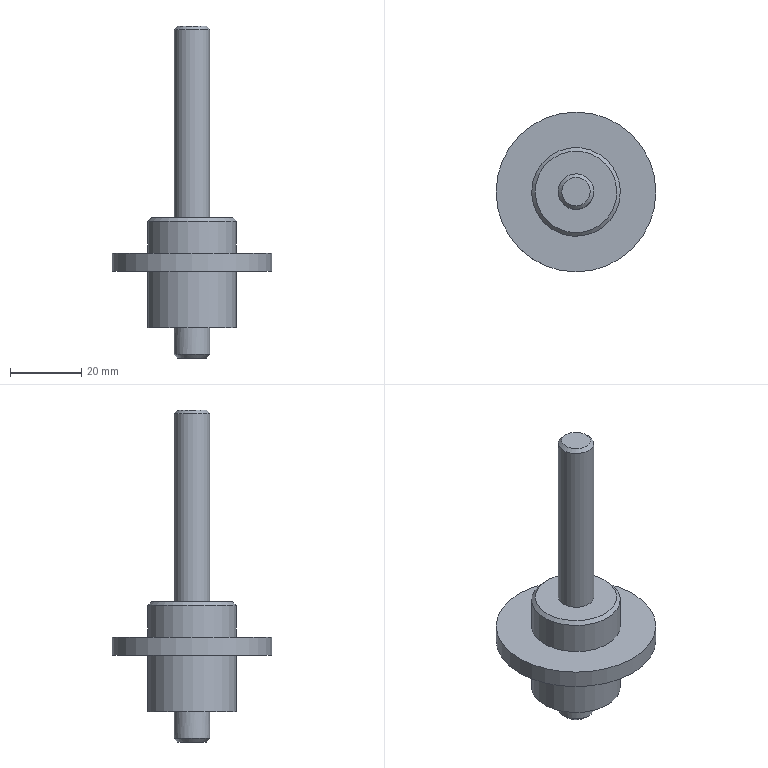Component | NX | MANDREL | 1 solid | 14 faces | box 45 x 45 x 93.5 mm | volume 25556 mm3 | plane 6 | cylinder 5 | cone 3 | commonest cylinder face diameters 25 x2 10 x2 45 x1
STEP:
#1=CARTESIAN_POINT('',(0.,0.,0.));
#2=DIRECTION('',(0.,0.,1.));
#3=DIRECTION('',(1.,0.,0.));
#4=AXIS2_PLACEMENT_3D('',#1,#2,#3);
#5=CARTESIAN_POINT('',(94.615,72.307,11.));
#6=VERTEX_POINT('',#5);
#7=CARTESIAN_POINT('',(89.996,70.391,11.));
#8=DIRECTION('',(0.,0.,-1.));
#9=DIRECTION('',(0.9237,0.383,0.));
#10=AXIS2_PLACEMENT_3D('',#7,#8,#9);
#11=CIRCLE('',#10,5.);
#12=CARTESIAN_POINT('',(89.996,70.391,11.));
#13=DIRECTION('',(0.,0.,1.));
#14=DIRECTION('',(0.383,-0.9237,0.));
#15=AXIS2_PLACEMENT_3D('',#12,#13,#14);
#16=PLANE('',#15);
#17=CARTESIAN_POINT('',(-0.,5.));
#18=CARTESIAN_POINT('',(8.66,5.));
#19=CARTESIAN_POINT('',(4.33,-2.5));
#20=CARTESIAN_POINT('',(0.,-10.));
#21=CARTESIAN_POINT('',(-4.33,-2.5));
#22=CARTESIAN_POINT('',(-8.66,5.));
#23=CARTESIAN_POINT('',(-0.,5.));
#24=(BOUNDED_CURVE()B_SPLINE_CURVE(2,(#17,#18,#19,#20,#21,#22,#23),.UNSPECIFIED.,.T.,.F.)B_SPLINE_CURVE_WITH_KNOTS((1,2,2,2,2,1),(-2.094,0.,2.094,4.189,6.283,8.378),.UNSPECIFIED.)CURVE()GEOMETRIC_REPRESENTATION_ITEM()RATIONAL_B_SPLINE_CURVE((1.,0.5,1.,0.5,1.,0.5,1.))REPRESENTATION_ITEM(''));
#25=(GEOMETRIC_REPRESENTATION_CONTEXT(2)PARAMETRIC_REPRESENTATION_CONTEXT()REPRESENTATION_CONTEXT('',''));
#26=DEFINITIONAL_REPRESENTATION('',(#24),#25);
#27=PCURVE('',#16,#26);
#28=CARTESIAN_POINT('',(89.996,70.391,2.5));
#29=DIRECTION('',(0.,0.,1.));
#30=DIRECTION('',(0.383,-0.9237,0.));
#31=AXIS2_PLACEMENT_3D('',#28,#29,#30);
#32=CYLINDRICAL_SURFACE('',#31,5.);
#33=CARTESIAN_POINT('',(7.854,8.5));
#34=DIRECTION('',(-1.,0.));
#35=VECTOR('',#34,1.);
#36=LINE('',#33,#35);
#37=(GEOMETRIC_REPRESENTATION_CONTEXT(2)PARAMETRIC_REPRESENTATION_CONTEXT()REPRESENTATION_CONTEXT('',''));
#38=DEFINITIONAL_REPRESENTATION('',(#36),#37);
#39=PCURVE('',#32,#38);
#40=SURFACE_CURVE('',#11,(#27,#39),.PCURVE_S1.);
#41=EDGE_CURVE('',#6,#6,#40,.T.);
#42=ORIENTED_EDGE('',*,*,#41,.F.);
#43=EDGE_LOOP('',(#42));
#44=FACE_BOUND('',#43,.T.);
#45=CARTESIAN_POINT('',(94.784,58.845,11.));
#46=VERTEX_POINT('',#45);
#47=CARTESIAN_POINT('',(89.996,70.391,11.));
#48=DIRECTION('',(0.,0.,1.));
#49=DIRECTION('',(0.383,-0.9237,0.));
#50=AXIS2_PLACEMENT_3D('',#47,#48,#49);
#51=CIRCLE('',#50,12.5);
#52=CARTESIAN_POINT('',(0.,0.));
#53=DIRECTION('',(1.,0.));
#54=AXIS2_PLACEMENT_2D('',#52,#53);
#55=CIRCLE('',#54,12.5);
#56=(GEOMETRIC_REPRESENTATION_CONTEXT(2)PARAMETRIC_REPRESENTATION_CONTEXT()REPRESENTATION_CONTEXT('',''));
#57=DEFINITIONAL_REPRESENTATION('',(#55),#56);
#58=PCURVE('',#16,#57);
#59=CARTESIAN_POINT('',(89.996,70.391,11.));
#60=DIRECTION('',(0.,0.,1.));
#61=DIRECTION('',(0.383,-0.9237,0.));
#62=AXIS2_PLACEMENT_3D('',#59,#60,#61);
#63=CYLINDRICAL_SURFACE('',#62,12.5);
#64=CARTESIAN_POINT('',(0.,0.));
#65=DIRECTION('',(1.,0.));
#66=VECTOR('',#65,1.);
#67=LINE('',#64,#66);
#68=(GEOMETRIC_REPRESENTATION_CONTEXT(2)PARAMETRIC_REPRESENTATION_CONTEXT()REPRESENTATION_CONTEXT('',''));
#69=DEFINITIONAL_REPRESENTATION('',(#67),#68);
#70=PCURVE('',#63,#69);
#71=SURFACE_CURVE('',#51,(#58,#70),.PCURVE_S1.);
#72=EDGE_CURVE('',#46,#46,#71,.T.);
#73=ORIENTED_EDGE('',*,*,#72,.F.);
#74=EDGE_LOOP('',(#73));
#75=FACE_BOUND('',#74,.T.);
#76=ADVANCED_FACE('',(#44,#75),#16,.F.);
#77=CARTESIAN_POINT('',(94.784,58.845,27.));
#78=VERTEX_POINT('',#77);
#79=CARTESIAN_POINT('',(89.996,70.391,27.));
#80=DIRECTION('',(0.,0.,1.));
#81=DIRECTION('',(0.383,-0.9237,0.));
#82=AXIS2_PLACEMENT_3D('',#79,#80,#81);
#83=CIRCLE('',#82,12.5);
#84=CARTESIAN_POINT('',(0.,16.));
#85=DIRECTION('',(1.,0.));
#86=VECTOR('',#85,1.);
#87=LINE('',#84,#86);
#88=(GEOMETRIC_REPRESENTATION_CONTEXT(2)PARAMETRIC_REPRESENTATION_CONTEXT()REPRESENTATION_CONTEXT('',''));
#89=DEFINITIONAL_REPRESENTATION('',(#87),#88);
#90=PCURVE('',#63,#89);
#91=CARTESIAN_POINT('',(85.208,81.938,27.));
#92=DIRECTION('',(0.,0.,1.));
#93=DIRECTION('',(0.383,-0.9237,0.));
#94=AXIS2_PLACEMENT_3D('',#91,#92,#93);
#95=PLANE('',#94);
#96=CARTESIAN_POINT('',(12.5,-0.));
#97=DIRECTION('',(1.,0.));
#98=AXIS2_PLACEMENT_2D('',#96,#97);
#99=CIRCLE('',#98,12.5);
#100=(GEOMETRIC_REPRESENTATION_CONTEXT(2)PARAMETRIC_REPRESENTATION_CONTEXT()REPRESENTATION_CONTEXT('',''));
#101=DEFINITIONAL_REPRESENTATION('',(#99),#100);
#102=PCURVE('',#95,#101);
#103=SURFACE_CURVE('',#83,(#90,#102),.PCURVE_S1.);
#104=EDGE_CURVE('',#78,#78,#103,.T.);
#105=ORIENTED_EDGE('',*,*,#104,.F.);
#106=CARTESIAN_POINT('',(94.784,58.845,11.));
#107=CARTESIAN_POINT('',(94.784,58.845,27.));
#108=B_SPLINE_CURVE_WITH_KNOTS('',1,(#106,#107),.UNSPECIFIED.,.F.,.F.,(2,2),(0.,16.),.PIECEWISE_BEZIER_KNOTS.);
#109=CARTESIAN_POINT('',(0.,0.));
#110=DIRECTION('',(0.,1.));
#111=VECTOR('',#110,1.);
#112=LINE('',#109,#111);
#113=(GEOMETRIC_REPRESENTATION_CONTEXT(2)PARAMETRIC_REPRESENTATION_CONTEXT()REPRESENTATION_CONTEXT('',''));
#114=DEFINITIONAL_REPRESENTATION('',(#112),#113);
#115=PCURVE('',#63,#114);
#116=CARTESIAN_POINT('',(6.283,0.));
#117=DIRECTION('',(0.,1.));
#118=VECTOR('',#117,1.);
#119=LINE('',#116,#118);
#120=(GEOMETRIC_REPRESENTATION_CONTEXT(2)PARAMETRIC_REPRESENTATION_CONTEXT()REPRESENTATION_CONTEXT('',''));
#121=DEFINITIONAL_REPRESENTATION('',(#119),#120);
#122=PCURVE('',#63,#121);
#123=SEAM_CURVE('',#108,(#115,#122),.PCURVE_S1.);
#124=EDGE_CURVE('',#46,#78,#123,.T.);
#125=ORIENTED_EDGE('',*,*,#124,.F.);
#126=ORIENTED_EDGE('',*,*,#72,.T.);
#127=ORIENTED_EDGE('',*,*,#124,.T.);
#128=EDGE_LOOP('',(#105,#125,#126,#127));
#129=FACE_BOUND('',#128,.T.);
#130=ADVANCED_FACE('',(#129),#63,.T.);
#131=CARTESIAN_POINT('',(98.615,49.608,27.));
#132=VERTEX_POINT('',#131);
#133=CARTESIAN_POINT('',(89.996,70.391,27.));
#134=DIRECTION('',(0.,0.,1.));
#135=DIRECTION('',(0.383,-0.9237,0.));
#136=AXIS2_PLACEMENT_3D('',#133,#134,#135);
#137=CIRCLE('',#136,22.5);
#138=CARTESIAN_POINT('',(12.5,-0.));
#139=DIRECTION('',(1.,0.));
#140=AXIS2_PLACEMENT_2D('',#138,#139);
#141=CIRCLE('',#140,22.5);
#142=(GEOMETRIC_REPRESENTATION_CONTEXT(2)PARAMETRIC_REPRESENTATION_CONTEXT()REPRESENTATION_CONTEXT('',''));
#143=DEFINITIONAL_REPRESENTATION('',(#141),#142);
#144=PCURVE('',#95,#143);
#145=CARTESIAN_POINT('',(89.996,70.391,11.));
#146=DIRECTION('',(0.,0.,1.));
#147=DIRECTION('',(0.383,-0.9237,0.));
#148=AXIS2_PLACEMENT_3D('',#145,#146,#147);
#149=CYLINDRICAL_SURFACE('',#148,22.5);
#150=CARTESIAN_POINT('',(0.,16.));
#151=DIRECTION('',(1.,0.));
#152=VECTOR('',#151,1.);
#153=LINE('',#150,#152);
#154=(GEOMETRIC_REPRESENTATION_CONTEXT(2)PARAMETRIC_REPRESENTATION_CONTEXT()REPRESENTATION_CONTEXT('',''));
#155=DEFINITIONAL_REPRESENTATION('',(#153),#154);
#156=PCURVE('',#149,#155);
#157=SURFACE_CURVE('',#137,(#144,#156),.PCURVE_S1.);
#158=EDGE_CURVE('',#132,#132,#157,.T.);
#159=ORIENTED_EDGE('',*,*,#158,.F.);
#160=EDGE_LOOP('',(#159));
#161=FACE_BOUND('',#160,.T.);
#162=ORIENTED_EDGE('',*,*,#104,.T.);
#163=EDGE_LOOP('',(#162));
#164=FACE_BOUND('',#163,.T.);
#165=ADVANCED_FACE('',(#161,#164),#95,.F.);
#166=CARTESIAN_POINT('',(98.615,49.608,32.));
#167=VERTEX_POINT('',#166);
#168=CARTESIAN_POINT('',(89.996,70.391,32.));
#169=DIRECTION('',(0.,0.,1.));
#170=DIRECTION('',(0.383,-0.9237,0.));
#171=AXIS2_PLACEMENT_3D('',#168,#169,#170);
#172=CIRCLE('',#171,22.5);
#173=CARTESIAN_POINT('',(0.,21.));
#174=DIRECTION('',(1.,0.));
#175=VECTOR('',#174,1.);
#176=LINE('',#173,#175);
#177=(GEOMETRIC_REPRESENTATION_CONTEXT(2)PARAMETRIC_REPRESENTATION_CONTEXT()REPRESENTATION_CONTEXT('',''));
#178=DEFINITIONAL_REPRESENTATION('',(#176),#177);
#179=PCURVE('',#149,#178);
#180=CARTESIAN_POINT('',(81.377,91.175,32.));
#181=DIRECTION('',(0.,0.,-1.));
#182=DIRECTION('',(-0.383,0.9237,0.));
#183=AXIS2_PLACEMENT_3D('',#180,#181,#182);
#184=PLANE('',#183);
#185=CARTESIAN_POINT('',(-45.,-0.));
#186=CARTESIAN_POINT('',(-45.,38.971));
#187=CARTESIAN_POINT('',(-11.25,19.486));
#188=CARTESIAN_POINT('',(22.5,-0.));
#189=CARTESIAN_POINT('',(-11.25,-19.486));
#190=CARTESIAN_POINT('',(-45.,-38.971));
#191=CARTESIAN_POINT('',(-45.,-0.));
#192=(BOUNDED_CURVE()B_SPLINE_CURVE(2,(#185,#186,#187,#188,#189,#190,#191),.UNSPECIFIED.,.T.,.F.)B_SPLINE_CURVE_WITH_KNOTS((1,2,2,2,2,1),(-2.094,0.,2.094,4.189,6.283,8.378),.UNSPECIFIED.)CURVE()GEOMETRIC_REPRESENTATION_ITEM()RATIONAL_B_SPLINE_CURVE((1.,0.5,1.,0.5,1.,0.5,1.))REPRESENTATION_ITEM(''));
#193=(GEOMETRIC_REPRESENTATION_CONTEXT(2)PARAMETRIC_REPRESENTATION_CONTEXT()REPRESENTATION_CONTEXT('',''));
#194=DEFINITIONAL_REPRESENTATION('',(#192),#193);
#195=PCURVE('',#184,#194);
#196=SURFACE_CURVE('',#172,(#179,#195),.PCURVE_S1.);
#197=EDGE_CURVE('',#167,#167,#196,.T.);
#198=ORIENTED_EDGE('',*,*,#197,.F.);
#199=CARTESIAN_POINT('',(98.615,49.608,27.));
#200=CARTESIAN_POINT('',(98.615,49.608,32.));
#201=B_SPLINE_CURVE_WITH_KNOTS('',1,(#199,#200),.UNSPECIFIED.,.F.,.F.,(2,2),(16.,21.),.PIECEWISE_BEZIER_KNOTS.);
#202=CARTESIAN_POINT('',(0.,0.));
#203=DIRECTION('',(0.,1.));
#204=VECTOR('',#203,1.);
#205=LINE('',#202,#204);
#206=(GEOMETRIC_REPRESENTATION_CONTEXT(2)PARAMETRIC_REPRESENTATION_CONTEXT()REPRESENTATION_CONTEXT('',''));
#207=DEFINITIONAL_REPRESENTATION('',(#205),#206);
#208=PCURVE('',#149,#207);
#209=CARTESIAN_POINT('',(6.283,0.));
#210=DIRECTION('',(0.,1.));
#211=VECTOR('',#210,1.);
#212=LINE('',#209,#211);
#213=(GEOMETRIC_REPRESENTATION_CONTEXT(2)PARAMETRIC_REPRESENTATION_CONTEXT()REPRESENTATION_CONTEXT('',''));
#214=DEFINITIONAL_REPRESENTATION('',(#212),#213);
#215=PCURVE('',#149,#214);
#216=SEAM_CURVE('',#201,(#208,#215),.PCURVE_S1.);
#217=EDGE_CURVE('',#132,#167,#216,.T.);
#218=ORIENTED_EDGE('',*,*,#217,.F.);
#219=ORIENTED_EDGE('',*,*,#158,.T.);
#220=ORIENTED_EDGE('',*,*,#217,.T.);
#221=EDGE_LOOP('',(#198,#218,#219,#220));
#222=FACE_BOUND('',#221,.T.);
#223=ADVANCED_FACE('',(#222),#149,.T.);
#224=CARTESIAN_POINT('',(94.784,58.845,32.));
#225=VERTEX_POINT('',#224);
#226=CARTESIAN_POINT('',(89.996,70.391,32.));
#227=DIRECTION('',(0.,0.,1.));
#228=DIRECTION('',(0.383,-0.9237,0.));
#229=AXIS2_PLACEMENT_3D('',#226,#227,#228);
#230=CIRCLE('',#229,12.5);
#231=CARTESIAN_POINT('',(-35.,-0.));
#232=CARTESIAN_POINT('',(-35.,21.651));
#233=CARTESIAN_POINT('',(-16.25,10.825));
#234=CARTESIAN_POINT('',(2.5,-0.));
#235=CARTESIAN_POINT('',(-16.25,-10.825));
#236=CARTESIAN_POINT('',(-35.,-21.651));
#237=CARTESIAN_POINT('',(-35.,-0.));
#238=(BOUNDED_CURVE()B_SPLINE_CURVE(2,(#231,#232,#233,#234,#235,#236,#237),.UNSPECIFIED.,.T.,.F.)B_SPLINE_CURVE_WITH_KNOTS((1,2,2,2,2,1),(-2.094,0.,2.094,4.189,6.283,8.378),.UNSPECIFIED.)CURVE()GEOMETRIC_REPRESENTATION_ITEM()RATIONAL_B_SPLINE_CURVE((1.,0.5,1.,0.5,1.,0.5,1.))REPRESENTATION_ITEM(''));
#239=(GEOMETRIC_REPRESENTATION_CONTEXT(2)PARAMETRIC_REPRESENTATION_CONTEXT()REPRESENTATION_CONTEXT('',''));
#240=DEFINITIONAL_REPRESENTATION('',(#238),#239);
#241=PCURVE('',#184,#240);
#242=CARTESIAN_POINT('',(89.996,70.391,11.));
#243=DIRECTION('',(0.,0.,1.));
#244=DIRECTION('',(0.383,-0.9237,0.));
#245=AXIS2_PLACEMENT_3D('',#242,#243,#244);
#246=CYLINDRICAL_SURFACE('',#245,12.5);
#247=CARTESIAN_POINT('',(0.,21.));
#248=DIRECTION('',(1.,0.));
#249=VECTOR('',#248,1.);
#250=LINE('',#247,#249);
#251=(GEOMETRIC_REPRESENTATION_CONTEXT(2)PARAMETRIC_REPRESENTATION_CONTEXT()REPRESENTATION_CONTEXT('',''));
#252=DEFINITIONAL_REPRESENTATION('',(#250),#251);
#253=PCURVE('',#246,#252);
#254=SURFACE_CURVE('',#230,(#241,#253),.PCURVE_S1.);
#255=EDGE_CURVE('',#225,#225,#254,.T.);
#256=ORIENTED_EDGE('',*,*,#255,.F.);
#257=EDGE_LOOP('',(#256));
#258=FACE_BOUND('',#257,.T.);
#259=ORIENTED_EDGE('',*,*,#197,.T.);
#260=EDGE_LOOP('',(#259));
#261=FACE_BOUND('',#260,.T.);
#262=ADVANCED_FACE('',(#258,#261),#184,.F.);
#263=CARTESIAN_POINT('',(85.208,81.938,41.));
#264=VERTEX_POINT('',#263);
#265=CARTESIAN_POINT('',(94.784,58.845,41.));
#266=VERTEX_POINT('',#265);
#267=CARTESIAN_POINT('',(89.996,70.391,41.));
#268=DIRECTION('',(0.,0.,-1.));
#269=DIRECTION('',(-0.383,0.9237,0.));
#270=AXIS2_PLACEMENT_3D('',#267,#268,#269);
#271=CIRCLE('',#270,12.5);
#272=CARTESIAN_POINT('',(3.142,30.));
#273=DIRECTION('',(-1.,0.));
#274=VECTOR('',#273,1.);
#275=LINE('',#272,#274);
#276=(GEOMETRIC_REPRESENTATION_CONTEXT(2)PARAMETRIC_REPRESENTATION_CONTEXT()REPRESENTATION_CONTEXT('',''));
#277=DEFINITIONAL_REPRESENTATION('',(#275),#276);
#278=PCURVE('',#246,#277);
#279=CARTESIAN_POINT('',(89.996,70.391,42.));
#280=DIRECTION('',(0.,0.,-1.));
#281=DIRECTION('',(-0.383,0.9237,0.));
#282=AXIS2_PLACEMENT_3D('',#279,#280,#281);
#283=CONICAL_SURFACE('',#282,11.5,0.7854);
#284=CARTESIAN_POINT('',(0.,1.));
#285=DIRECTION('',(1.,-0.));
#286=VECTOR('',#285,1.);
#287=LINE('',#284,#286);
#288=(GEOMETRIC_REPRESENTATION_CONTEXT(2)PARAMETRIC_REPRESENTATION_CONTEXT()REPRESENTATION_CONTEXT('',''));
#289=DEFINITIONAL_REPRESENTATION('',(#287),#288);
#290=PCURVE('',#283,#289);
#291=SURFACE_CURVE('',#271,(#278,#290),.PCURVE_S1.);
#292=EDGE_CURVE('',#264,#266,#291,.T.);
#293=ORIENTED_EDGE('',*,*,#292,.T.);
#294=CARTESIAN_POINT('',(94.784,58.845,32.));
#295=CARTESIAN_POINT('',(94.784,58.845,41.));
#296=B_SPLINE_CURVE_WITH_KNOTS('',1,(#294,#295),.UNSPECIFIED.,.F.,.F.,(2,2),(21.,30.),.PIECEWISE_BEZIER_KNOTS.);
#297=CARTESIAN_POINT('',(0.,0.));
#298=DIRECTION('',(0.,1.));
#299=VECTOR('',#298,1.);
#300=LINE('',#297,#299);
#301=(GEOMETRIC_REPRESENTATION_CONTEXT(2)PARAMETRIC_REPRESENTATION_CONTEXT()REPRESENTATION_CONTEXT('',''));
#302=DEFINITIONAL_REPRESENTATION('',(#300),#301);
#303=PCURVE('',#246,#302);
#304=CARTESIAN_POINT('',(6.283,0.));
#305=DIRECTION('',(0.,1.));
#306=VECTOR('',#305,1.);
#307=LINE('',#304,#306);
#308=(GEOMETRIC_REPRESENTATION_CONTEXT(2)PARAMETRIC_REPRESENTATION_CONTEXT()REPRESENTATION_CONTEXT('',''));
#309=DEFINITIONAL_REPRESENTATION('',(#307),#308);
#310=PCURVE('',#246,#309);
#311=SEAM_CURVE('',#296,(#303,#310),.PCURVE_S1.);
#312=EDGE_CURVE('',#225,#266,#311,.T.);
#313=ORIENTED_EDGE('',*,*,#312,.F.);
#314=ORIENTED_EDGE('',*,*,#255,.T.);
#315=ORIENTED_EDGE('',*,*,#312,.T.);
#316=CARTESIAN_POINT('',(89.996,70.391,41.));
#317=DIRECTION('',(0.,0.,-1.));
#318=DIRECTION('',(-0.383,0.9237,0.));
#319=AXIS2_PLACEMENT_3D('',#316,#317,#318);
#320=CIRCLE('',#319,12.5);
#321=CARTESIAN_POINT('',(9.425,30.));
#322=DIRECTION('',(-1.,0.));
#323=VECTOR('',#322,1.);
#324=LINE('',#321,#323);
#325=(GEOMETRIC_REPRESENTATION_CONTEXT(2)PARAMETRIC_REPRESENTATION_CONTEXT()REPRESENTATION_CONTEXT('',''));
#326=DEFINITIONAL_REPRESENTATION('',(#324),#325);
#327=PCURVE('',#246,#326);
#328=CARTESIAN_POINT('',(0.,1.));
#329=DIRECTION('',(1.,0.));
#330=VECTOR('',#329,1.);
#331=LINE('',#328,#330);
#332=(GEOMETRIC_REPRESENTATION_CONTEXT(2)PARAMETRIC_REPRESENTATION_CONTEXT()REPRESENTATION_CONTEXT('',''));
#333=DEFINITIONAL_REPRESENTATION('',(#331),#332);
#334=PCURVE('',#283,#333);
#335=SURFACE_CURVE('',#320,(#327,#334),.PCURVE_S1.);
#336=EDGE_CURVE('',#266,#264,#335,.T.);
#337=ORIENTED_EDGE('',*,*,#336,.T.);
#338=EDGE_LOOP('',(#293,#313,#314,#315,#337));
#339=FACE_BOUND('',#338,.T.);
#340=ADVANCED_FACE('',(#339),#246,.T.);
#341=CARTESIAN_POINT('',(85.591,81.014,42.));
#342=VERTEX_POINT('',#341);
#343=CARTESIAN_POINT('',(89.996,70.391,42.));
#344=DIRECTION('',(0.,0.,1.));
#345=DIRECTION('',(-0.383,0.9237,0.));
#346=AXIS2_PLACEMENT_3D('',#343,#344,#345);
#347=CIRCLE('',#346,11.5);
#348=CARTESIAN_POINT('',(85.208,81.938,42.));
#349=DIRECTION('',(0.,0.,-1.));
#350=DIRECTION('',(-0.383,0.9237,0.));
#351=AXIS2_PLACEMENT_3D('',#348,#349,#350);
#352=PLANE('',#351);
#353=CARTESIAN_POINT('',(-1.,0.));
#354=CARTESIAN_POINT('',(-1.,-19.919));
#355=CARTESIAN_POINT('',(-18.25,-9.959));
#356=CARTESIAN_POINT('',(-35.5,-0.));
#357=CARTESIAN_POINT('',(-18.25,9.959));
#358=CARTESIAN_POINT('',(-1.,19.919));
#359=CARTESIAN_POINT('',(-1.,0.));
#360=(BOUNDED_CURVE()B_SPLINE_CURVE(2,(#353,#354,#355,#356,#357,#358,#359),.UNSPECIFIED.,.T.,.F.)B_SPLINE_CURVE_WITH_KNOTS((1,2,2,2,2,1),(-2.094,0.,2.094,4.189,6.283,8.378),.UNSPECIFIED.)CURVE()GEOMETRIC_REPRESENTATION_ITEM()RATIONAL_B_SPLINE_CURVE((1.,0.5,1.,0.5,1.,0.5,1.))REPRESENTATION_ITEM(''));
#361=(GEOMETRIC_REPRESENTATION_CONTEXT(2)PARAMETRIC_REPRESENTATION_CONTEXT()REPRESENTATION_CONTEXT('',''));
#362=DEFINITIONAL_REPRESENTATION('',(#360),#361);
#363=PCURVE('',#352,#362);
#364=CARTESIAN_POINT('',(6.283,0.));
#365=DIRECTION('',(-1.,0.));
#366=VECTOR('',#365,1.);
#367=LINE('',#364,#366);
#368=(GEOMETRIC_REPRESENTATION_CONTEXT(2)PARAMETRIC_REPRESENTATION_CONTEXT()REPRESENTATION_CONTEXT('',''));
#369=DEFINITIONAL_REPRESENTATION('',(#367),#368);
#370=PCURVE('',#283,#369);
#371=SURFACE_CURVE('',#347,(#363,#370),.PCURVE_S1.);
#372=EDGE_CURVE('',#342,#342,#371,.T.);
#373=ORIENTED_EDGE('',*,*,#372,.T.);
#374=EDGE_LOOP('',(#373));
#375=FACE_BOUND('',#374,.T.);
#376=CARTESIAN_POINT('',(91.911,65.773,42.));
#377=VERTEX_POINT('',#376);
#378=CARTESIAN_POINT('',(89.996,70.391,42.));
#379=DIRECTION('',(0.,0.,1.));
#380=DIRECTION('',(0.383,-0.9237,0.));
#381=AXIS2_PLACEMENT_3D('',#378,#379,#380);
#382=CIRCLE('',#381,5.);
#383=CARTESIAN_POINT('',(-17.5,0.));
#384=CARTESIAN_POINT('',(-17.5,8.66));
#385=CARTESIAN_POINT('',(-10.,4.33));
#386=CARTESIAN_POINT('',(-2.5,-0.));
#387=CARTESIAN_POINT('',(-10.,-4.33));
#388=CARTESIAN_POINT('',(-17.5,-8.66));
#389=CARTESIAN_POINT('',(-17.5,0.));
#390=(BOUNDED_CURVE()B_SPLINE_CURVE(2,(#383,#384,#385,#386,#387,#388,#389),.UNSPECIFIED.,.T.,.F.)B_SPLINE_CURVE_WITH_KNOTS((1,2,2,2,2,1),(-2.094,0.,2.094,4.189,6.283,8.378),.UNSPECIFIED.)CURVE()GEOMETRIC_REPRESENTATION_ITEM()RATIONAL_B_SPLINE_CURVE((1.,0.5,1.,0.5,1.,0.5,1.))REPRESENTATION_ITEM(''));
#391=(GEOMETRIC_REPRESENTATION_CONTEXT(2)PARAMETRIC_REPRESENTATION_CONTEXT()REPRESENTATION_CONTEXT('',''));
#392=DEFINITIONAL_REPRESENTATION('',(#390),#391);
#393=PCURVE('',#352,#392);
#394=CARTESIAN_POINT('',(89.996,70.391,11.));
#395=DIRECTION('',(0.,0.,1.));
#396=DIRECTION('',(0.383,-0.9237,0.));
#397=AXIS2_PLACEMENT_3D('',#394,#395,#396);
#398=CYLINDRICAL_SURFACE('',#397,5.);
#399=CARTESIAN_POINT('',(0.,31.));
#400=DIRECTION('',(1.,0.));
#401=VECTOR('',#400,1.);
#402=LINE('',#399,#401);
#403=(GEOMETRIC_REPRESENTATION_CONTEXT(2)PARAMETRIC_REPRESENTATION_CONTEXT()REPRESENTATION_CONTEXT('',''));
#404=DEFINITIONAL_REPRESENTATION('',(#402),#403);
#405=PCURVE('',#398,#404);
#406=SURFACE_CURVE('',#382,(#393,#405),.PCURVE_S1.);
#407=EDGE_CURVE('',#377,#377,#406,.T.);
#408=ORIENTED_EDGE('',*,*,#407,.F.);
#409=EDGE_LOOP('',(#408));
#410=FACE_BOUND('',#409,.T.);
#411=ADVANCED_FACE('',(#375,#410),#352,.F.);
#412=CARTESIAN_POINT('',(88.081,75.01,95.));
#413=VERTEX_POINT('',#412);
#414=CARTESIAN_POINT('',(91.911,65.773,95.));
#415=VERTEX_POINT('',#414);
#416=CARTESIAN_POINT('',(89.996,70.391,95.));
#417=DIRECTION('',(0.,0.,-1.));
#418=DIRECTION('',(-0.383,0.9237,0.));
#419=AXIS2_PLACEMENT_3D('',#416,#417,#418);
#420=CIRCLE('',#419,5.);
#421=CARTESIAN_POINT('',(3.142,84.));
#422=DIRECTION('',(-1.,0.));
#423=VECTOR('',#422,1.);
#424=LINE('',#421,#423);
#425=(GEOMETRIC_REPRESENTATION_CONTEXT(2)PARAMETRIC_REPRESENTATION_CONTEXT()REPRESENTATION_CONTEXT('',''));
#426=DEFINITIONAL_REPRESENTATION('',(#424),#425);
#427=PCURVE('',#398,#426);
#428=CARTESIAN_POINT('',(89.996,70.391,96.));
#429=DIRECTION('',(0.,0.,-1.));
#430=DIRECTION('',(-0.383,0.9237,0.));
#431=AXIS2_PLACEMENT_3D('',#428,#429,#430);
#432=CONICAL_SURFACE('',#431,4.,0.7854);
#433=CARTESIAN_POINT('',(0.,1.));
#434=DIRECTION('',(1.,-0.));
#435=VECTOR('',#434,1.);
#436=LINE('',#433,#435);
#437=(GEOMETRIC_REPRESENTATION_CONTEXT(2)PARAMETRIC_REPRESENTATION_CONTEXT()REPRESENTATION_CONTEXT('',''));
#438=DEFINITIONAL_REPRESENTATION('',(#436),#437);
#439=PCURVE('',#432,#438);
#440=SURFACE_CURVE('',#420,(#427,#439),.PCURVE_S1.);
#441=EDGE_CURVE('',#413,#415,#440,.T.);
#442=ORIENTED_EDGE('',*,*,#441,.T.);
#443=CARTESIAN_POINT('',(91.911,65.773,42.));
#444=CARTESIAN_POINT('',(91.911,65.773,95.));
#445=B_SPLINE_CURVE_WITH_KNOTS('',1,(#443,#444),.UNSPECIFIED.,.F.,.F.,(2,2),(31.,84.),.PIECEWISE_BEZIER_KNOTS.);
#446=CARTESIAN_POINT('',(0.,0.));
#447=DIRECTION('',(0.,1.));
#448=VECTOR('',#447,1.);
#449=LINE('',#446,#448);
#450=(GEOMETRIC_REPRESENTATION_CONTEXT(2)PARAMETRIC_REPRESENTATION_CONTEXT()REPRESENTATION_CONTEXT('',''));
#451=DEFINITIONAL_REPRESENTATION('',(#449),#450);
#452=PCURVE('',#398,#451);
#453=CARTESIAN_POINT('',(6.283,0.));
#454=DIRECTION('',(0.,1.));
#455=VECTOR('',#454,1.);
#456=LINE('',#453,#455);
#457=(GEOMETRIC_REPRESENTATION_CONTEXT(2)PARAMETRIC_REPRESENTATION_CONTEXT()REPRESENTATION_CONTEXT('',''));
#458=DEFINITIONAL_REPRESENTATION('',(#456),#457);
#459=PCURVE('',#398,#458);
#460=SEAM_CURVE('',#445,(#452,#459),.PCURVE_S1.);
#461=EDGE_CURVE('',#377,#415,#460,.T.);
#462=ORIENTED_EDGE('',*,*,#461,.F.);
#463=ORIENTED_EDGE('',*,*,#407,.T.);
#464=ORIENTED_EDGE('',*,*,#461,.T.);
#465=CARTESIAN_POINT('',(89.996,70.391,95.));
#466=DIRECTION('',(0.,0.,-1.));
#467=DIRECTION('',(-0.383,0.9237,0.));
#468=AXIS2_PLACEMENT_3D('',#465,#466,#467);
#469=CIRCLE('',#468,5.);
#470=CARTESIAN_POINT('',(9.425,84.));
#471=DIRECTION('',(-1.,0.));
#472=VECTOR('',#471,1.);
#473=LINE('',#470,#472);
#474=(GEOMETRIC_REPRESENTATION_CONTEXT(2)PARAMETRIC_REPRESENTATION_CONTEXT()REPRESENTATION_CONTEXT('',''));
#475=DEFINITIONAL_REPRESENTATION('',(#473),#474);
#476=PCURVE('',#398,#475);
#477=CARTESIAN_POINT('',(-0.,1.));
#478=DIRECTION('',(1.,0.));
#479=VECTOR('',#478,1.);
#480=LINE('',#477,#479);
#481=(GEOMETRIC_REPRESENTATION_CONTEXT(2)PARAMETRIC_REPRESENTATION_CONTEXT()REPRESENTATION_CONTEXT('',''));
#482=DEFINITIONAL_REPRESENTATION('',(#480),#481);
#483=PCURVE('',#432,#482);
#484=SURFACE_CURVE('',#469,(#476,#483),.PCURVE_S1.);
#485=EDGE_CURVE('',#415,#413,#484,.T.);
#486=ORIENTED_EDGE('',*,*,#485,.T.);
#487=EDGE_LOOP('',(#442,#462,#463,#464,#486));
#488=FACE_BOUND('',#487,.T.);
#489=ADVANCED_FACE('',(#488),#398,.T.);
#490=CARTESIAN_POINT('',(88.464,74.086,96.));
#491=VERTEX_POINT('',#490);
#492=CARTESIAN_POINT('',(89.996,70.391,96.));
#493=DIRECTION('',(0.,0.,1.));
#494=DIRECTION('',(-0.383,0.9237,0.));
#495=AXIS2_PLACEMENT_3D('',#492,#493,#494);
#496=CIRCLE('',#495,4.);
#497=CARTESIAN_POINT('',(88.081,75.01,96.));
#498=DIRECTION('',(0.,0.,-1.));
#499=DIRECTION('',(-0.383,0.9237,0.));
#500=AXIS2_PLACEMENT_3D('',#497,#498,#499);
#501=PLANE('',#500);
#502=CARTESIAN_POINT('',(-1.,-0.));
#503=CARTESIAN_POINT('',(-1.,-6.928));
#504=CARTESIAN_POINT('',(-7.,-3.464));
#505=CARTESIAN_POINT('',(-13.,-0.));
#506=CARTESIAN_POINT('',(-7.,3.464));
#507=CARTESIAN_POINT('',(-1.,6.928));
#508=CARTESIAN_POINT('',(-1.,-0.));
#509=(BOUNDED_CURVE()B_SPLINE_CURVE(2,(#502,#503,#504,#505,#506,#507,#508),.UNSPECIFIED.,.T.,.F.)B_SPLINE_CURVE_WITH_KNOTS((1,2,2,2,2,1),(-2.094,0.,2.094,4.189,6.283,8.378),.UNSPECIFIED.)CURVE()GEOMETRIC_REPRESENTATION_ITEM()RATIONAL_B_SPLINE_CURVE((1.,0.5,1.,0.5,1.,0.5,1.))REPRESENTATION_ITEM(''));
#510=(GEOMETRIC_REPRESENTATION_CONTEXT(2)PARAMETRIC_REPRESENTATION_CONTEXT()REPRESENTATION_CONTEXT('',''));
#511=DEFINITIONAL_REPRESENTATION('',(#509),#510);
#512=PCURVE('',#501,#511);
#513=CARTESIAN_POINT('',(6.283,-0.));
#514=DIRECTION('',(-1.,0.));
#515=VECTOR('',#514,1.);
#516=LINE('',#513,#515);
#517=(GEOMETRIC_REPRESENTATION_CONTEXT(2)PARAMETRIC_REPRESENTATION_CONTEXT()REPRESENTATION_CONTEXT('',''));
#518=DEFINITIONAL_REPRESENTATION('',(#516),#517);
#519=PCURVE('',#432,#518);
#520=SURFACE_CURVE('',#496,(#512,#519),.PCURVE_S1.);
#521=EDGE_CURVE('',#491,#491,#520,.T.);
#522=ORIENTED_EDGE('',*,*,#521,.T.);
#523=EDGE_LOOP('',(#522));
#524=FACE_BOUND('',#523,.T.);
#525=ADVANCED_FACE('',(#524),#501,.F.);
#526=CARTESIAN_POINT('',(88.081,75.01,3.5));
#527=VERTEX_POINT('',#526);
#528=CARTESIAN_POINT('',(94.615,72.307,3.5));
#529=VERTEX_POINT('',#528);
#530=CARTESIAN_POINT('',(89.996,70.391,3.5));
#531=DIRECTION('',(0.,0.,1.));
#532=DIRECTION('',(-0.383,0.9237,0.));
#533=AXIS2_PLACEMENT_3D('',#530,#531,#532);
#534=CIRCLE('',#533,5.);
#535=CARTESIAN_POINT('',(3.142,1.));
#536=DIRECTION('',(1.,0.));
#537=VECTOR('',#536,1.);
#538=LINE('',#535,#537);
#539=(GEOMETRIC_REPRESENTATION_CONTEXT(2)PARAMETRIC_REPRESENTATION_CONTEXT()REPRESENTATION_CONTEXT('',''));
#540=DEFINITIONAL_REPRESENTATION('',(#538),#539);
#541=PCURVE('',#32,#540);
#542=CARTESIAN_POINT('',(89.996,70.391,2.5));
#543=DIRECTION('',(0.,0.,1.));
#544=DIRECTION('',(0.383,-0.9237,0.));
#545=AXIS2_PLACEMENT_3D('',#542,#543,#544);
#546=CONICAL_SURFACE('',#545,4.,0.7854);
#547=CARTESIAN_POINT('',(3.142,1.));
#548=DIRECTION('',(1.,-0.));
#549=VECTOR('',#548,1.);
#550=LINE('',#547,#549);
#551=(GEOMETRIC_REPRESENTATION_CONTEXT(2)PARAMETRIC_REPRESENTATION_CONTEXT()REPRESENTATION_CONTEXT('',''));
#552=DEFINITIONAL_REPRESENTATION('',(#550),#551);
#553=PCURVE('',#546,#552);
#554=SURFACE_CURVE('',#534,(#541,#553),.PCURVE_S1.);
#555=EDGE_CURVE('',#527,#529,#554,.T.);
#556=ORIENTED_EDGE('',*,*,#555,.T.);
#557=CARTESIAN_POINT('',(94.615,72.307,3.5));
#558=CARTESIAN_POINT('',(94.615,72.307,11.));
#559=B_SPLINE_CURVE_WITH_KNOTS('',1,(#557,#558),.UNSPECIFIED.,.F.,.F.,(2,2),(1.,8.5),.PIECEWISE_BEZIER_KNOTS.);
#560=CARTESIAN_POINT('',(7.854,0.));
#561=DIRECTION('',(0.,1.));
#562=VECTOR('',#561,1.);
#563=LINE('',#560,#562);
#564=(GEOMETRIC_REPRESENTATION_CONTEXT(2)PARAMETRIC_REPRESENTATION_CONTEXT()REPRESENTATION_CONTEXT('',''));
#565=DEFINITIONAL_REPRESENTATION('',(#563),#564);
#566=PCURVE('',#32,#565);
#567=CARTESIAN_POINT('',(1.571,0.));
#568=DIRECTION('',(0.,1.));
#569=VECTOR('',#568,1.);
#570=LINE('',#567,#569);
#571=(GEOMETRIC_REPRESENTATION_CONTEXT(2)PARAMETRIC_REPRESENTATION_CONTEXT()REPRESENTATION_CONTEXT('',''));
#572=DEFINITIONAL_REPRESENTATION('',(#570),#571);
#573=PCURVE('',#32,#572);
#574=SEAM_CURVE('',#559,(#566,#573),.PCURVE_S1.);
#575=EDGE_CURVE('',#529,#6,#574,.T.);
#576=ORIENTED_EDGE('',*,*,#575,.T.);
#577=ORIENTED_EDGE('',*,*,#41,.T.);
#578=ORIENTED_EDGE('',*,*,#575,.F.);
#579=CARTESIAN_POINT('',(89.996,70.391,3.5));
#580=DIRECTION('',(0.,0.,1.));
#581=DIRECTION('',(-0.383,0.9237,0.));
#582=AXIS2_PLACEMENT_3D('',#579,#580,#581);
#583=CIRCLE('',#582,5.);
#584=CARTESIAN_POINT('',(-3.142,1.));
#585=DIRECTION('',(1.,0.));
#586=VECTOR('',#585,1.);
#587=LINE('',#584,#586);
#588=(GEOMETRIC_REPRESENTATION_CONTEXT(2)PARAMETRIC_REPRESENTATION_CONTEXT()REPRESENTATION_CONTEXT('',''));
#589=DEFINITIONAL_REPRESENTATION('',(#587),#588);
#590=PCURVE('',#32,#589);
#591=CARTESIAN_POINT('',(3.142,1.));
#592=DIRECTION('',(1.,0.));
#593=VECTOR('',#592,1.);
#594=LINE('',#591,#593);
#595=(GEOMETRIC_REPRESENTATION_CONTEXT(2)PARAMETRIC_REPRESENTATION_CONTEXT()REPRESENTATION_CONTEXT('',''));
#596=DEFINITIONAL_REPRESENTATION('',(#594),#595);
#597=PCURVE('',#546,#596);
#598=SURFACE_CURVE('',#583,(#590,#597),.PCURVE_S1.);
#599=EDGE_CURVE('',#529,#527,#598,.T.);
#600=ORIENTED_EDGE('',*,*,#599,.T.);
#601=EDGE_LOOP('',(#556,#576,#577,#578,#600));
#602=FACE_BOUND('',#601,.T.);
#603=ADVANCED_FACE('',(#602),#32,.T.);
#604=CARTESIAN_POINT('',(88.464,74.086,2.5));
#605=VERTEX_POINT('',#604);
#606=CARTESIAN_POINT('',(89.996,70.391,2.5));
#607=DIRECTION('',(0.,0.,-1.));
#608=DIRECTION('',(-0.383,0.9237,0.));
#609=AXIS2_PLACEMENT_3D('',#606,#607,#608);
#610=CIRCLE('',#609,4.);
#611=CARTESIAN_POINT('',(89.996,70.391,2.5));
#612=DIRECTION('',(0.,0.,-1.));
#613=DIRECTION('',(-0.383,0.9237,0.));
#614=AXIS2_PLACEMENT_3D('',#611,#612,#613);
#615=PLANE('',#614);
#616=CARTESIAN_POINT('',(0.,0.));
#617=DIRECTION('',(1.,0.));
#618=AXIS2_PLACEMENT_2D('',#616,#617);
#619=CIRCLE('',#618,4.);
#620=(GEOMETRIC_REPRESENTATION_CONTEXT(2)PARAMETRIC_REPRESENTATION_CONTEXT()REPRESENTATION_CONTEXT('',''));
#621=DEFINITIONAL_REPRESENTATION('',(#619),#620);
#622=PCURVE('',#615,#621);
#623=CARTESIAN_POINT('',(9.425,-0.));
#624=DIRECTION('',(-1.,0.));
#625=VECTOR('',#624,1.);
#626=LINE('',#623,#625);
#627=(GEOMETRIC_REPRESENTATION_CONTEXT(2)PARAMETRIC_REPRESENTATION_CONTEXT()REPRESENTATION_CONTEXT('',''));
#628=DEFINITIONAL_REPRESENTATION('',(#626),#627);
#629=PCURVE('',#546,#628);
#630=SURFACE_CURVE('',#610,(#622,#629),.PCURVE_S1.);
#631=EDGE_CURVE('',#605,#605,#630,.T.);
#632=ORIENTED_EDGE('',*,*,#631,.T.);
#633=EDGE_LOOP('',(#632));
#634=FACE_BOUND('',#633,.T.);
#635=ADVANCED_FACE('',(#634),#615,.T.);
#636=ORIENTED_EDGE('',*,*,#441,.F.);
#637=CARTESIAN_POINT('',(88.464,74.086,96.));
#638=CARTESIAN_POINT('',(88.081,75.01,95.));
#639=B_SPLINE_CURVE_WITH_KNOTS('',1,(#637,#638),.UNSPECIFIED.,.F.,.F.,(2,2),(-0.,1.414),.PIECEWISE_BEZIER_KNOTS.);
#640=CARTESIAN_POINT('',(0.,0.));
#641=DIRECTION('',(0.,1.));
#642=VECTOR('',#641,1.);
#643=LINE('',#640,#642);
#644=(GEOMETRIC_REPRESENTATION_CONTEXT(2)PARAMETRIC_REPRESENTATION_CONTEXT()REPRESENTATION_CONTEXT('',''));
#645=DEFINITIONAL_REPRESENTATION('',(#643),#644);
#646=PCURVE('',#432,#645);
#647=CARTESIAN_POINT('',(6.283,0.));
#648=DIRECTION('',(0.,1.));
#649=VECTOR('',#648,1.);
#650=LINE('',#647,#649);
#651=(GEOMETRIC_REPRESENTATION_CONTEXT(2)PARAMETRIC_REPRESENTATION_CONTEXT()REPRESENTATION_CONTEXT('',''));
#652=DEFINITIONAL_REPRESENTATION('',(#650),#651);
#653=PCURVE('',#432,#652);
#654=SEAM_CURVE('',#639,(#646,#653),.PCURVE_S1.);
#655=EDGE_CURVE('',#491,#413,#654,.T.);
#656=ORIENTED_EDGE('',*,*,#655,.F.);
#657=ORIENTED_EDGE('',*,*,#521,.F.);
#658=ORIENTED_EDGE('',*,*,#655,.T.);
#659=ORIENTED_EDGE('',*,*,#485,.F.);
#660=EDGE_LOOP('',(#636,#656,#657,#658,#659));
#661=FACE_BOUND('',#660,.T.);
#662=ADVANCED_FACE('',(#661),#432,.T.);
#663=ORIENTED_EDGE('',*,*,#292,.F.);
#664=CARTESIAN_POINT('',(85.591,81.014,42.));
#665=CARTESIAN_POINT('',(85.208,81.938,41.));
#666=B_SPLINE_CURVE_WITH_KNOTS('',1,(#664,#665),.UNSPECIFIED.,.F.,.F.,(2,2),(0.,1.414),.PIECEWISE_BEZIER_KNOTS.);
#667=CARTESIAN_POINT('',(0.,0.));
#668=DIRECTION('',(0.,1.));
#669=VECTOR('',#668,1.);
#670=LINE('',#667,#669);
#671=(GEOMETRIC_REPRESENTATION_CONTEXT(2)PARAMETRIC_REPRESENTATION_CONTEXT()REPRESENTATION_CONTEXT('',''));
#672=DEFINITIONAL_REPRESENTATION('',(#670),#671);
#673=PCURVE('',#283,#672);
#674=CARTESIAN_POINT('',(6.283,0.));
#675=DIRECTION('',(0.,1.));
#676=VECTOR('',#675,1.);
#677=LINE('',#674,#676);
#678=(GEOMETRIC_REPRESENTATION_CONTEXT(2)PARAMETRIC_REPRESENTATION_CONTEXT()REPRESENTATION_CONTEXT('',''));
#679=DEFINITIONAL_REPRESENTATION('',(#677),#678);
#680=PCURVE('',#283,#679);
#681=SEAM_CURVE('',#666,(#673,#680),.PCURVE_S1.);
#682=EDGE_CURVE('',#342,#264,#681,.T.);
#683=ORIENTED_EDGE('',*,*,#682,.F.);
#684=ORIENTED_EDGE('',*,*,#372,.F.);
#685=ORIENTED_EDGE('',*,*,#682,.T.);
#686=ORIENTED_EDGE('',*,*,#336,.F.);
#687=EDGE_LOOP('',(#663,#683,#684,#685,#686));
#688=FACE_BOUND('',#687,.T.);
#689=ADVANCED_FACE('',(#688),#283,.T.);
#690=ORIENTED_EDGE('',*,*,#555,.F.);
#691=CARTESIAN_POINT('',(88.464,74.086,2.5));
#692=CARTESIAN_POINT('',(88.081,75.01,3.5));
#693=B_SPLINE_CURVE_WITH_KNOTS('',1,(#691,#692),.UNSPECIFIED.,.F.,.F.,(2,2),(-0.,1.414),.PIECEWISE_BEZIER_KNOTS.);
#694=CARTESIAN_POINT('',(3.142,0.));
#695=DIRECTION('',(0.,1.));
#696=VECTOR('',#695,1.);
#697=LINE('',#694,#696);
#698=(GEOMETRIC_REPRESENTATION_CONTEXT(2)PARAMETRIC_REPRESENTATION_CONTEXT()REPRESENTATION_CONTEXT('',''));
#699=DEFINITIONAL_REPRESENTATION('',(#697),#698);
#700=PCURVE('',#546,#699);
#701=CARTESIAN_POINT('',(9.425,0.));
#702=DIRECTION('',(0.,1.));
#703=VECTOR('',#702,1.);
#704=LINE('',#701,#703);
#705=(GEOMETRIC_REPRESENTATION_CONTEXT(2)PARAMETRIC_REPRESENTATION_CONTEXT()REPRESENTATION_CONTEXT('',''));
#706=DEFINITIONAL_REPRESENTATION('',(#704),#705);
#707=PCURVE('',#546,#706);
#708=SEAM_CURVE('',#693,(#700,#707),.PCURVE_S1.);
#709=EDGE_CURVE('',#605,#527,#708,.T.);
#710=ORIENTED_EDGE('',*,*,#709,.F.);
#711=ORIENTED_EDGE('',*,*,#631,.F.);
#712=ORIENTED_EDGE('',*,*,#709,.T.);
#713=ORIENTED_EDGE('',*,*,#599,.F.);
#714=EDGE_LOOP('',(#690,#710,#711,#712,#713));
#715=FACE_BOUND('',#714,.T.);
#716=ADVANCED_FACE('',(#715),#546,.T.);
#717=CLOSED_SHELL('',(#76,#130,#165,#223,#262,#340,#411,#489,#525,#603,#635,#662,#689,#716));
#718=MANIFOLD_SOLID_BREP('',#717);
#719=(LENGTH_UNIT()NAMED_UNIT(*)SI_UNIT(.MILLI.,.METRE.));
#720=UNCERTAINTY_MEASURE_WITH_UNIT(LENGTH_MEASURE(0.00001),#719,'','');
#721=(NAMED_UNIT(*)PLANE_ANGLE_UNIT()SI_UNIT($,.RADIAN.));
#722=(NAMED_UNIT(*)SI_UNIT($,.STERADIAN.)SOLID_ANGLE_UNIT());
#723=(GEOMETRIC_REPRESENTATION_CONTEXT(3)GLOBAL_UNCERTAINTY_ASSIGNED_CONTEXT((#720))GLOBAL_UNIT_ASSIGNED_CONTEXT((#719,#721,#722))REPRESENTATION_CONTEXT('',''));
#724=ADVANCED_BREP_SHAPE_REPRESENTATION('',(#4,#718),#723);